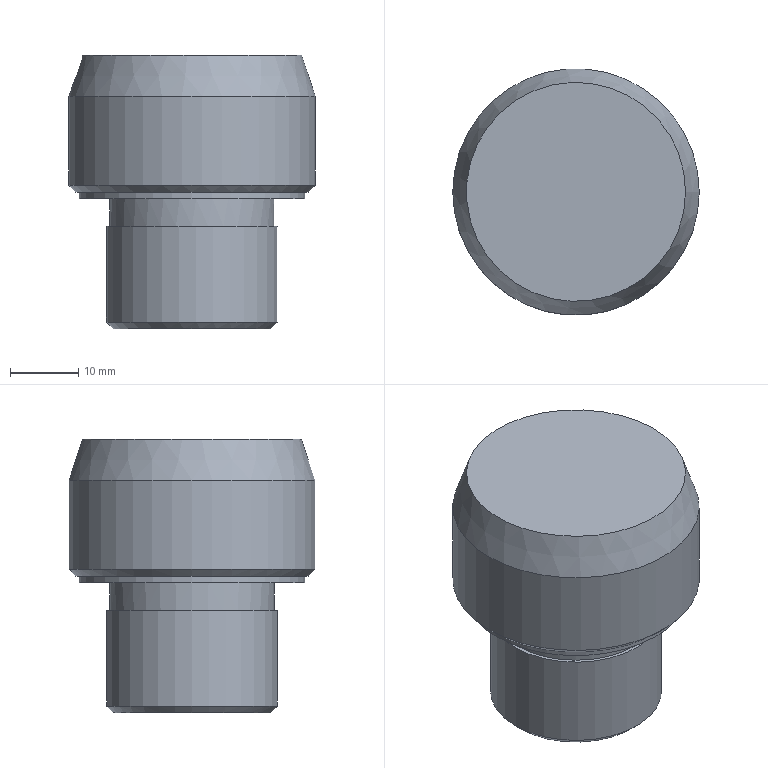Component | NX | CYL_LOC_PIN | 1 solid | 12 faces | box 36 x 36 x 40 mm | volume 29638 mm3 | plane 5 | cylinder 4 | cone 3 | commonest cylinder face diameters 36 x1 33 x1 24 x1 25 x1
STEP:
#1=CARTESIAN_POINT('',(0.,0.,0.));
#2=DIRECTION('',(0.,0.,1.));
#3=DIRECTION('',(1.,0.,0.));
#4=AXIS2_PLACEMENT_3D('',#1,#2,#3);
#5=CARTESIAN_POINT('',(-105.,0.,-236.));
#6=VERTEX_POINT('',#5);
#7=CARTESIAN_POINT('',(-88.,0.,-236.));
#8=DIRECTION('',(0.,0.,-1.));
#9=DIRECTION('',(-1.,0.,0.));
#10=AXIS2_PLACEMENT_3D('',#7,#8,#9);
#11=CIRCLE('',#10,17.);
#12=CARTESIAN_POINT('',(-88.,0.,-236.));
#13=DIRECTION('',(0.,0.,-1.));
#14=DIRECTION('',(-1.,0.,0.));
#15=AXIS2_PLACEMENT_3D('',#12,#13,#14);
#16=PLANE('',#15);
#17=CARTESIAN_POINT('',(0.,0.));
#18=DIRECTION('',(1.,0.));
#19=AXIS2_PLACEMENT_2D('',#17,#18);
#20=CIRCLE('',#19,17.);
#21=(GEOMETRIC_REPRESENTATION_CONTEXT(2)PARAMETRIC_REPRESENTATION_CONTEXT()REPRESENTATION_CONTEXT('',''));
#22=DEFINITIONAL_REPRESENTATION('',(#20),#21);
#23=PCURVE('',#16,#22);
#24=CARTESIAN_POINT('',(-88.,0.,-235.));
#25=DIRECTION('',(0.,0.,1.));
#26=DIRECTION('',(1.,0.,0.));
#27=AXIS2_PLACEMENT_3D('',#24,#25,#26);
#28=CONICAL_SURFACE('',#27,18.,0.7854);
#29=CARTESIAN_POINT('',(9.425,-1.));
#30=DIRECTION('',(-1.,0.));
#31=VECTOR('',#30,1.);
#32=LINE('',#29,#31);
#33=(GEOMETRIC_REPRESENTATION_CONTEXT(2)PARAMETRIC_REPRESENTATION_CONTEXT()REPRESENTATION_CONTEXT('',''));
#34=DEFINITIONAL_REPRESENTATION('',(#32),#33);
#35=PCURVE('',#28,#34);
#36=SURFACE_CURVE('',#11,(#23,#35),.PCURVE_S1.);
#37=EDGE_CURVE('',#6,#6,#36,.T.);
#38=ORIENTED_EDGE('',*,*,#37,.T.);
#39=EDGE_LOOP('',(#38));
#40=FACE_BOUND('',#39,.T.);
#41=CARTESIAN_POINT('',(-104.5,0.,-236.));
#42=VERTEX_POINT('',#41);
#43=CARTESIAN_POINT('',(-88.,0.,-236.));
#44=DIRECTION('',(0.,0.,-1.));
#45=DIRECTION('',(-1.,0.,0.));
#46=AXIS2_PLACEMENT_3D('',#43,#44,#45);
#47=CIRCLE('',#46,16.5);
#48=CARTESIAN_POINT('',(0.,0.));
#49=DIRECTION('',(1.,0.));
#50=AXIS2_PLACEMENT_2D('',#48,#49);
#51=CIRCLE('',#50,16.5);
#52=(GEOMETRIC_REPRESENTATION_CONTEXT(2)PARAMETRIC_REPRESENTATION_CONTEXT()REPRESENTATION_CONTEXT('',''));
#53=DEFINITIONAL_REPRESENTATION('',(#51),#52);
#54=PCURVE('',#16,#53);
#55=CARTESIAN_POINT('',(-88.,0.,-236.));
#56=DIRECTION('',(0.,0.,-1.));
#57=DIRECTION('',(-1.,0.,0.));
#58=AXIS2_PLACEMENT_3D('',#55,#56,#57);
#59=CYLINDRICAL_SURFACE('',#58,16.5);
#60=CARTESIAN_POINT('',(0.,0.));
#61=DIRECTION('',(1.,0.));
#62=VECTOR('',#61,1.);
#63=LINE('',#60,#62);
#64=(GEOMETRIC_REPRESENTATION_CONTEXT(2)PARAMETRIC_REPRESENTATION_CONTEXT()REPRESENTATION_CONTEXT('',''));
#65=DEFINITIONAL_REPRESENTATION('',(#63),#64);
#66=PCURVE('',#59,#65);
#67=SURFACE_CURVE('',#47,(#54,#66),.PCURVE_S1.);
#68=EDGE_CURVE('',#42,#42,#67,.T.);
#69=ORIENTED_EDGE('',*,*,#68,.F.);
#70=EDGE_LOOP('',(#69));
#71=FACE_BOUND('',#70,.T.);
#72=ADVANCED_FACE('',(#40,#71),#16,.T.);
#73=CARTESIAN_POINT('',(-72.,0.,-216.));
#74=VERTEX_POINT('',#73);
#75=CARTESIAN_POINT('',(-88.,0.,-216.));
#76=DIRECTION('',(0.,0.,1.));
#77=DIRECTION('',(1.,0.,0.));
#78=AXIS2_PLACEMENT_3D('',#75,#76,#77);
#79=CIRCLE('',#78,16.);
#80=CARTESIAN_POINT('',(-88.,0.,-216.));
#81=DIRECTION('',(0.,0.,1.));
#82=DIRECTION('',(1.,0.,0.));
#83=AXIS2_PLACEMENT_3D('',#80,#81,#82);
#84=PLANE('',#83);
#85=CARTESIAN_POINT('',(0.,0.));
#86=DIRECTION('',(1.,0.));
#87=AXIS2_PLACEMENT_2D('',#85,#86);
#88=CIRCLE('',#87,16.);
#89=(GEOMETRIC_REPRESENTATION_CONTEXT(2)PARAMETRIC_REPRESENTATION_CONTEXT()REPRESENTATION_CONTEXT('',''));
#90=DEFINITIONAL_REPRESENTATION('',(#88),#89);
#91=PCURVE('',#84,#90);
#92=CARTESIAN_POINT('',(-88.,0.,-222.));
#93=DIRECTION('',(0.,0.,-1.));
#94=DIRECTION('',(-1.,0.,0.));
#95=AXIS2_PLACEMENT_3D('',#92,#93,#94);
#96=CONICAL_SURFACE('',#95,18.,0.3218);
#97=CARTESIAN_POINT('',(9.425,-6.));
#98=DIRECTION('',(-1.,0.));
#99=VECTOR('',#98,1.);
#100=LINE('',#97,#99);
#101=(GEOMETRIC_REPRESENTATION_CONTEXT(2)PARAMETRIC_REPRESENTATION_CONTEXT()REPRESENTATION_CONTEXT('',''));
#102=DEFINITIONAL_REPRESENTATION('',(#100),#101);
#103=PCURVE('',#96,#102);
#104=SURFACE_CURVE('',#79,(#91,#103),.PCURVE_S1.);
#105=EDGE_CURVE('',#74,#74,#104,.T.);
#106=ORIENTED_EDGE('',*,*,#105,.T.);
#107=EDGE_LOOP('',(#106));
#108=FACE_BOUND('',#107,.T.);
#109=ADVANCED_FACE('',(#108),#84,.T.);
#110=CARTESIAN_POINT('',(-106.,0.,-235.));
#111=VERTEX_POINT('',#110);
#112=CARTESIAN_POINT('',(-88.,0.,-235.));
#113=DIRECTION('',(0.,0.,1.));
#114=DIRECTION('',(-1.,0.,0.));
#115=AXIS2_PLACEMENT_3D('',#112,#113,#114);
#116=CIRCLE('',#115,18.);
#117=CARTESIAN_POINT('',(-88.,0.,-216.));
#118=DIRECTION('',(0.,0.,-1.));
#119=DIRECTION('',(-1.,0.,0.));
#120=AXIS2_PLACEMENT_3D('',#117,#118,#119);
#121=CYLINDRICAL_SURFACE('',#120,18.);
#122=CARTESIAN_POINT('',(6.283,19.));
#123=DIRECTION('',(-1.,0.));
#124=VECTOR('',#123,1.);
#125=LINE('',#122,#124);
#126=(GEOMETRIC_REPRESENTATION_CONTEXT(2)PARAMETRIC_REPRESENTATION_CONTEXT()REPRESENTATION_CONTEXT('',''));
#127=DEFINITIONAL_REPRESENTATION('',(#125),#126);
#128=PCURVE('',#121,#127);
#129=CARTESIAN_POINT('',(3.142,0.));
#130=DIRECTION('',(1.,0.));
#131=VECTOR('',#130,1.);
#132=LINE('',#129,#131);
#133=(GEOMETRIC_REPRESENTATION_CONTEXT(2)PARAMETRIC_REPRESENTATION_CONTEXT()REPRESENTATION_CONTEXT('',''));
#134=DEFINITIONAL_REPRESENTATION('',(#132),#133);
#135=PCURVE('',#28,#134);
#136=SURFACE_CURVE('',#116,(#128,#135),.PCURVE_S1.);
#137=EDGE_CURVE('',#111,#111,#136,.T.);
#138=ORIENTED_EDGE('',*,*,#137,.T.);
#139=CARTESIAN_POINT('',(-106.,0.,-222.));
#140=VERTEX_POINT('',#139);
#141=CARTESIAN_POINT('',(-106.,0.,-222.));
#142=CARTESIAN_POINT('',(-106.,0.,-235.));
#143=B_SPLINE_CURVE_WITH_KNOTS('',1,(#141,#142),.UNSPECIFIED.,.F.,.F.,(2,2),(6.,19.),.PIECEWISE_BEZIER_KNOTS.);
#144=CARTESIAN_POINT('',(0.,0.));
#145=DIRECTION('',(0.,1.));
#146=VECTOR('',#145,1.);
#147=LINE('',#144,#146);
#148=(GEOMETRIC_REPRESENTATION_CONTEXT(2)PARAMETRIC_REPRESENTATION_CONTEXT()REPRESENTATION_CONTEXT('',''));
#149=DEFINITIONAL_REPRESENTATION('',(#147),#148);
#150=PCURVE('',#121,#149);
#151=CARTESIAN_POINT('',(6.283,0.));
#152=DIRECTION('',(0.,1.));
#153=VECTOR('',#152,1.);
#154=LINE('',#151,#153);
#155=(GEOMETRIC_REPRESENTATION_CONTEXT(2)PARAMETRIC_REPRESENTATION_CONTEXT()REPRESENTATION_CONTEXT('',''));
#156=DEFINITIONAL_REPRESENTATION('',(#154),#155);
#157=PCURVE('',#121,#156);
#158=SEAM_CURVE('',#143,(#150,#157),.PCURVE_S1.);
#159=EDGE_CURVE('',#140,#111,#158,.T.);
#160=ORIENTED_EDGE('',*,*,#159,.F.);
#161=CARTESIAN_POINT('',(-70.,0.,-222.));
#162=VERTEX_POINT('',#161);
#163=CARTESIAN_POINT('',(-88.,0.,-222.));
#164=DIRECTION('',(0.,0.,-1.));
#165=DIRECTION('',(1.,0.,0.));
#166=AXIS2_PLACEMENT_3D('',#163,#164,#165);
#167=CIRCLE('',#166,18.);
#168=CARTESIAN_POINT('',(-3.142,6.));
#169=DIRECTION('',(1.,0.));
#170=VECTOR('',#169,1.);
#171=LINE('',#168,#170);
#172=(GEOMETRIC_REPRESENTATION_CONTEXT(2)PARAMETRIC_REPRESENTATION_CONTEXT()REPRESENTATION_CONTEXT('',''));
#173=DEFINITIONAL_REPRESENTATION('',(#171),#172);
#174=PCURVE('',#121,#173);
#175=CARTESIAN_POINT('',(3.142,0.));
#176=DIRECTION('',(1.,0.));
#177=VECTOR('',#176,1.);
#178=LINE('',#175,#177);
#179=(GEOMETRIC_REPRESENTATION_CONTEXT(2)PARAMETRIC_REPRESENTATION_CONTEXT()REPRESENTATION_CONTEXT('',''));
#180=DEFINITIONAL_REPRESENTATION('',(#178),#179);
#181=PCURVE('',#96,#180);
#182=SURFACE_CURVE('',#167,(#174,#181),.PCURVE_S1.);
#183=EDGE_CURVE('',#140,#162,#182,.T.);
#184=ORIENTED_EDGE('',*,*,#183,.T.);
#185=CARTESIAN_POINT('',(-88.,0.,-222.));
#186=DIRECTION('',(0.,0.,-1.));
#187=DIRECTION('',(1.,0.,0.));
#188=AXIS2_PLACEMENT_3D('',#185,#186,#187);
#189=CIRCLE('',#188,18.);
#190=CARTESIAN_POINT('',(3.142,6.));
#191=DIRECTION('',(1.,0.));
#192=VECTOR('',#191,1.);
#193=LINE('',#190,#192);
#194=(GEOMETRIC_REPRESENTATION_CONTEXT(2)PARAMETRIC_REPRESENTATION_CONTEXT()REPRESENTATION_CONTEXT('',''));
#195=DEFINITIONAL_REPRESENTATION('',(#193),#194);
#196=PCURVE('',#121,#195);
#197=CARTESIAN_POINT('',(3.142,0.));
#198=DIRECTION('',(1.,0.));
#199=VECTOR('',#198,1.);
#200=LINE('',#197,#199);
#201=(GEOMETRIC_REPRESENTATION_CONTEXT(2)PARAMETRIC_REPRESENTATION_CONTEXT()REPRESENTATION_CONTEXT('',''));
#202=DEFINITIONAL_REPRESENTATION('',(#200),#201);
#203=PCURVE('',#96,#202);
#204=SURFACE_CURVE('',#189,(#196,#203),.PCURVE_S1.);
#205=EDGE_CURVE('',#162,#140,#204,.T.);
#206=ORIENTED_EDGE('',*,*,#205,.T.);
#207=ORIENTED_EDGE('',*,*,#159,.T.);
#208=EDGE_LOOP('',(#138,#160,#184,#206,#207));
#209=FACE_BOUND('',#208,.T.);
#210=ADVANCED_FACE('',(#209),#121,.T.);
#211=CARTESIAN_POINT('',(-100.,0.,-237.));
#212=VERTEX_POINT('',#211);
#213=CARTESIAN_POINT('',(-88.,0.,-237.));
#214=DIRECTION('',(0.,0.,-1.));
#215=DIRECTION('',(-1.,0.,0.));
#216=AXIS2_PLACEMENT_3D('',#213,#214,#215);
#217=CIRCLE('',#216,12.);
#218=CARTESIAN_POINT('',(-88.,0.,-237.));
#219=DIRECTION('',(0.,0.,-1.));
#220=DIRECTION('',(-1.,0.,0.));
#221=AXIS2_PLACEMENT_3D('',#218,#219,#220);
#222=PLANE('',#221);
#223=CARTESIAN_POINT('',(0.,0.));
#224=DIRECTION('',(1.,0.));
#225=AXIS2_PLACEMENT_2D('',#223,#224);
#226=CIRCLE('',#225,12.);
#227=(GEOMETRIC_REPRESENTATION_CONTEXT(2)PARAMETRIC_REPRESENTATION_CONTEXT()REPRESENTATION_CONTEXT('',''));
#228=DEFINITIONAL_REPRESENTATION('',(#226),#227);
#229=PCURVE('',#222,#228);
#230=CARTESIAN_POINT('',(-88.,0.,-237.));
#231=DIRECTION('',(0.,0.,-1.));
#232=DIRECTION('',(-1.,0.,0.));
#233=AXIS2_PLACEMENT_3D('',#230,#231,#232);
#234=CYLINDRICAL_SURFACE('',#233,12.);
#235=CARTESIAN_POINT('',(0.,0.));
#236=DIRECTION('',(1.,0.));
#237=VECTOR('',#236,1.);
#238=LINE('',#235,#237);
#239=(GEOMETRIC_REPRESENTATION_CONTEXT(2)PARAMETRIC_REPRESENTATION_CONTEXT()REPRESENTATION_CONTEXT('',''));
#240=DEFINITIONAL_REPRESENTATION('',(#238),#239);
#241=PCURVE('',#234,#240);
#242=SURFACE_CURVE('',#217,(#229,#241),.PCURVE_S1.);
#243=EDGE_CURVE('',#212,#212,#242,.T.);
#244=ORIENTED_EDGE('',*,*,#243,.F.);
#245=EDGE_LOOP('',(#244));
#246=FACE_BOUND('',#245,.T.);
#247=CARTESIAN_POINT('',(-104.5,0.,-237.));
#248=VERTEX_POINT('',#247);
#249=CARTESIAN_POINT('',(-88.,0.,-237.));
#250=DIRECTION('',(0.,0.,1.));
#251=DIRECTION('',(-1.,0.,0.));
#252=AXIS2_PLACEMENT_3D('',#249,#250,#251);
#253=CIRCLE('',#252,16.5);
#254=CARTESIAN_POINT('',(16.5,0.));
#255=CARTESIAN_POINT('',(16.5,-28.579));
#256=CARTESIAN_POINT('',(-8.25,-14.289));
#257=CARTESIAN_POINT('',(-33.,-0.));
#258=CARTESIAN_POINT('',(-8.25,14.289));
#259=CARTESIAN_POINT('',(16.5,28.579));
#260=CARTESIAN_POINT('',(16.5,0.));
#261=(BOUNDED_CURVE()B_SPLINE_CURVE(2,(#254,#255,#256,#257,#258,#259,#260),.UNSPECIFIED.,.T.,.F.)B_SPLINE_CURVE_WITH_KNOTS((1,2,2,2,2,1),(-2.094,0.,2.094,4.189,6.283,8.378),.UNSPECIFIED.)CURVE()GEOMETRIC_REPRESENTATION_ITEM()RATIONAL_B_SPLINE_CURVE((1.,0.5,1.,0.5,1.,0.5,1.))REPRESENTATION_ITEM(''));
#262=(GEOMETRIC_REPRESENTATION_CONTEXT(2)PARAMETRIC_REPRESENTATION_CONTEXT()REPRESENTATION_CONTEXT('',''));
#263=DEFINITIONAL_REPRESENTATION('',(#261),#262);
#264=PCURVE('',#222,#263);
#265=CARTESIAN_POINT('',(6.283,1.));
#266=DIRECTION('',(-1.,0.));
#267=VECTOR('',#266,1.);
#268=LINE('',#265,#267);
#269=(GEOMETRIC_REPRESENTATION_CONTEXT(2)PARAMETRIC_REPRESENTATION_CONTEXT()REPRESENTATION_CONTEXT('',''));
#270=DEFINITIONAL_REPRESENTATION('',(#268),#269);
#271=PCURVE('',#59,#270);
#272=SURFACE_CURVE('',#253,(#264,#271),.PCURVE_S1.);
#273=EDGE_CURVE('',#248,#248,#272,.T.);
#274=ORIENTED_EDGE('',*,*,#273,.F.);
#275=EDGE_LOOP('',(#274));
#276=FACE_BOUND('',#275,.T.);
#277=ADVANCED_FACE('',(#246,#276),#222,.T.);
#278=ORIENTED_EDGE('',*,*,#273,.T.);
#279=CARTESIAN_POINT('',(-104.5,0.,-236.));
#280=CARTESIAN_POINT('',(-104.5,0.,-237.));
#281=B_SPLINE_CURVE_WITH_KNOTS('',1,(#279,#280),.UNSPECIFIED.,.F.,.F.,(2,2),(0.,1.),.PIECEWISE_BEZIER_KNOTS.);
#282=CARTESIAN_POINT('',(0.,0.));
#283=DIRECTION('',(0.,1.));
#284=VECTOR('',#283,1.);
#285=LINE('',#282,#284);
#286=(GEOMETRIC_REPRESENTATION_CONTEXT(2)PARAMETRIC_REPRESENTATION_CONTEXT()REPRESENTATION_CONTEXT('',''));
#287=DEFINITIONAL_REPRESENTATION('',(#285),#286);
#288=PCURVE('',#59,#287);
#289=CARTESIAN_POINT('',(6.283,0.));
#290=DIRECTION('',(0.,1.));
#291=VECTOR('',#290,1.);
#292=LINE('',#289,#291);
#293=(GEOMETRIC_REPRESENTATION_CONTEXT(2)PARAMETRIC_REPRESENTATION_CONTEXT()REPRESENTATION_CONTEXT('',''));
#294=DEFINITIONAL_REPRESENTATION('',(#292),#293);
#295=PCURVE('',#59,#294);
#296=SEAM_CURVE('',#281,(#288,#295),.PCURVE_S1.);
#297=EDGE_CURVE('',#42,#248,#296,.T.);
#298=ORIENTED_EDGE('',*,*,#297,.F.);
#299=ORIENTED_EDGE('',*,*,#68,.T.);
#300=ORIENTED_EDGE('',*,*,#297,.T.);
#301=EDGE_LOOP('',(#278,#298,#299,#300));
#302=FACE_BOUND('',#301,.T.);
#303=ADVANCED_FACE('',(#302),#59,.T.);
#304=CARTESIAN_POINT('',(-100.,0.,-241.));
#305=VERTEX_POINT('',#304);
#306=CARTESIAN_POINT('',(-76.,0.,-241.));
#307=VERTEX_POINT('',#306);
#308=CARTESIAN_POINT('',(-88.,0.,-241.));
#309=DIRECTION('',(0.,0.,-1.));
#310=DIRECTION('',(1.,0.,0.));
#311=AXIS2_PLACEMENT_3D('',#308,#309,#310);
#312=CIRCLE('',#311,12.);
#313=CARTESIAN_POINT('',(-3.142,4.));
#314=DIRECTION('',(1.,0.));
#315=VECTOR('',#314,1.);
#316=LINE('',#313,#315);
#317=(GEOMETRIC_REPRESENTATION_CONTEXT(2)PARAMETRIC_REPRESENTATION_CONTEXT()REPRESENTATION_CONTEXT('',''));
#318=DEFINITIONAL_REPRESENTATION('',(#316),#317);
#319=PCURVE('',#234,#318);
#320=CARTESIAN_POINT('',(-88.,0.,-241.));
#321=DIRECTION('',(0.,0.,1.));
#322=DIRECTION('',(1.,0.,0.));
#323=AXIS2_PLACEMENT_3D('',#320,#321,#322);
#324=PLANE('',#323);
#325=CARTESIAN_POINT('',(12.,0.));
#326=CARTESIAN_POINT('',(12.,-20.785));
#327=CARTESIAN_POINT('',(-6.,-10.392));
#328=CARTESIAN_POINT('',(-24.,-0.));
#329=CARTESIAN_POINT('',(-6.,10.392));
#330=CARTESIAN_POINT('',(12.,20.785));
#331=CARTESIAN_POINT('',(12.,0.));
#332=(BOUNDED_CURVE()B_SPLINE_CURVE(2,(#325,#326,#327,#328,#329,#330,#331),.UNSPECIFIED.,.T.,.F.)B_SPLINE_CURVE_WITH_KNOTS((1,2,2,2,2,1),(-2.094,0.,2.094,4.189,6.283,8.378),.UNSPECIFIED.)CURVE()GEOMETRIC_REPRESENTATION_ITEM()RATIONAL_B_SPLINE_CURVE((1.,0.5,1.,0.5,1.,0.5,1.))REPRESENTATION_ITEM(''));
#333=(GEOMETRIC_REPRESENTATION_CONTEXT(2)PARAMETRIC_REPRESENTATION_CONTEXT()REPRESENTATION_CONTEXT('',''));
#334=DEFINITIONAL_REPRESENTATION('',(#332),#333);
#335=PCURVE('',#324,#334);
#336=SURFACE_CURVE('',#312,(#319,#335),.PCURVE_S1.);
#337=EDGE_CURVE('',#305,#307,#336,.T.);
#338=ORIENTED_EDGE('',*,*,#337,.F.);
#339=CARTESIAN_POINT('',(-100.,0.,-237.));
#340=CARTESIAN_POINT('',(-100.,0.,-241.));
#341=B_SPLINE_CURVE_WITH_KNOTS('',1,(#339,#340),.UNSPECIFIED.,.F.,.F.,(2,2),(0.,4.),.PIECEWISE_BEZIER_KNOTS.);
#342=CARTESIAN_POINT('',(0.,0.));
#343=DIRECTION('',(0.,1.));
#344=VECTOR('',#343,1.);
#345=LINE('',#342,#344);
#346=(GEOMETRIC_REPRESENTATION_CONTEXT(2)PARAMETRIC_REPRESENTATION_CONTEXT()REPRESENTATION_CONTEXT('',''));
#347=DEFINITIONAL_REPRESENTATION('',(#345),#346);
#348=PCURVE('',#234,#347);
#349=CARTESIAN_POINT('',(6.283,0.));
#350=DIRECTION('',(0.,1.));
#351=VECTOR('',#350,1.);
#352=LINE('',#349,#351);
#353=(GEOMETRIC_REPRESENTATION_CONTEXT(2)PARAMETRIC_REPRESENTATION_CONTEXT()REPRESENTATION_CONTEXT('',''));
#354=DEFINITIONAL_REPRESENTATION('',(#352),#353);
#355=PCURVE('',#234,#354);
#356=SEAM_CURVE('',#341,(#348,#355),.PCURVE_S1.);
#357=EDGE_CURVE('',#212,#305,#356,.T.);
#358=ORIENTED_EDGE('',*,*,#357,.F.);
#359=ORIENTED_EDGE('',*,*,#243,.T.);
#360=ORIENTED_EDGE('',*,*,#357,.T.);
#361=CARTESIAN_POINT('',(-88.,0.,-241.));
#362=DIRECTION('',(0.,0.,-1.));
#363=DIRECTION('',(1.,0.,0.));
#364=AXIS2_PLACEMENT_3D('',#361,#362,#363);
#365=CIRCLE('',#364,12.);
#366=CARTESIAN_POINT('',(3.142,4.));
#367=DIRECTION('',(1.,0.));
#368=VECTOR('',#367,1.);
#369=LINE('',#366,#368);
#370=(GEOMETRIC_REPRESENTATION_CONTEXT(2)PARAMETRIC_REPRESENTATION_CONTEXT()REPRESENTATION_CONTEXT('',''));
#371=DEFINITIONAL_REPRESENTATION('',(#369),#370);
#372=PCURVE('',#234,#371);
#373=CARTESIAN_POINT('',(12.,0.));
#374=CARTESIAN_POINT('',(12.,-20.785));
#375=CARTESIAN_POINT('',(-6.,-10.392));
#376=CARTESIAN_POINT('',(-24.,-0.));
#377=CARTESIAN_POINT('',(-6.,10.392));
#378=CARTESIAN_POINT('',(12.,20.785));
#379=CARTESIAN_POINT('',(12.,0.));
#380=(BOUNDED_CURVE()B_SPLINE_CURVE(2,(#373,#374,#375,#376,#377,#378,#379),.UNSPECIFIED.,.T.,.F.)B_SPLINE_CURVE_WITH_KNOTS((1,2,2,2,2,1),(-2.094,0.,2.094,4.189,6.283,8.378),.UNSPECIFIED.)CURVE()GEOMETRIC_REPRESENTATION_ITEM()RATIONAL_B_SPLINE_CURVE((1.,0.5,1.,0.5,1.,0.5,1.))REPRESENTATION_ITEM(''));
#381=(GEOMETRIC_REPRESENTATION_CONTEXT(2)PARAMETRIC_REPRESENTATION_CONTEXT()REPRESENTATION_CONTEXT('',''));
#382=DEFINITIONAL_REPRESENTATION('',(#380),#381);
#383=PCURVE('',#324,#382);
#384=SURFACE_CURVE('',#365,(#372,#383),.PCURVE_S1.);
#385=EDGE_CURVE('',#307,#305,#384,.T.);
#386=ORIENTED_EDGE('',*,*,#385,.F.);
#387=EDGE_LOOP('',(#338,#358,#359,#360,#386));
#388=FACE_BOUND('',#387,.T.);
#389=ADVANCED_FACE('',(#388),#234,.T.);
#390=CARTESIAN_POINT('',(-99.5,0.,-256.));
#391=VERTEX_POINT('',#390);
#392=CARTESIAN_POINT('',(-88.,0.,-256.));
#393=DIRECTION('',(0.,0.,-1.));
#394=DIRECTION('',(-1.,0.,0.));
#395=AXIS2_PLACEMENT_3D('',#392,#393,#394);
#396=CIRCLE('',#395,11.5);
#397=CARTESIAN_POINT('',(-88.,0.,-256.));
#398=DIRECTION('',(0.,0.,-1.));
#399=DIRECTION('',(-1.,0.,0.));
#400=AXIS2_PLACEMENT_3D('',#397,#398,#399);
#401=PLANE('',#400);
#402=CARTESIAN_POINT('',(0.,0.));
#403=DIRECTION('',(1.,0.));
#404=AXIS2_PLACEMENT_2D('',#402,#403);
#405=CIRCLE('',#404,11.5);
#406=(GEOMETRIC_REPRESENTATION_CONTEXT(2)PARAMETRIC_REPRESENTATION_CONTEXT()REPRESENTATION_CONTEXT('',''));
#407=DEFINITIONAL_REPRESENTATION('',(#405),#406);
#408=PCURVE('',#401,#407);
#409=CARTESIAN_POINT('',(-88.,0.,-255.));
#410=DIRECTION('',(0.,0.,1.));
#411=DIRECTION('',(1.,0.,0.));
#412=AXIS2_PLACEMENT_3D('',#409,#410,#411);
#413=CONICAL_SURFACE('',#412,12.5,0.7854);
#414=CARTESIAN_POINT('',(9.425,-1.));
#415=DIRECTION('',(-1.,0.));
#416=VECTOR('',#415,1.);
#417=LINE('',#414,#416);
#418=(GEOMETRIC_REPRESENTATION_CONTEXT(2)PARAMETRIC_REPRESENTATION_CONTEXT()REPRESENTATION_CONTEXT('',''));
#419=DEFINITIONAL_REPRESENTATION('',(#417),#418);
#420=PCURVE('',#413,#419);
#421=SURFACE_CURVE('',#396,(#408,#420),.PCURVE_S1.);
#422=EDGE_CURVE('',#391,#391,#421,.T.);
#423=ORIENTED_EDGE('',*,*,#422,.T.);
#424=EDGE_LOOP('',(#423));
#425=FACE_BOUND('',#424,.T.);
#426=ADVANCED_FACE('',(#425),#401,.T.);
#427=ORIENTED_EDGE('',*,*,#385,.T.);
#428=ORIENTED_EDGE('',*,*,#337,.T.);
#429=EDGE_LOOP('',(#427,#428));
#430=FACE_BOUND('',#429,.T.);
#431=CARTESIAN_POINT('',(-100.5,0.,-241.));
#432=VERTEX_POINT('',#431);
#433=CARTESIAN_POINT('',(-88.,0.,-241.));
#434=DIRECTION('',(0.,0.,-1.));
#435=DIRECTION('',(-1.,0.,0.));
#436=AXIS2_PLACEMENT_3D('',#433,#434,#435);
#437=CIRCLE('',#436,12.5);
#438=CARTESIAN_POINT('',(-12.5,0.));
#439=CARTESIAN_POINT('',(-12.5,21.651));
#440=CARTESIAN_POINT('',(6.25,10.825));
#441=CARTESIAN_POINT('',(25.,0.));
#442=CARTESIAN_POINT('',(6.25,-10.825));
#443=CARTESIAN_POINT('',(-12.5,-21.651));
#444=CARTESIAN_POINT('',(-12.5,0.));
#445=(BOUNDED_CURVE()B_SPLINE_CURVE(2,(#438,#439,#440,#441,#442,#443,#444),.UNSPECIFIED.,.T.,.F.)B_SPLINE_CURVE_WITH_KNOTS((1,2,2,2,2,1),(-2.094,0.,2.094,4.189,6.283,8.378),.UNSPECIFIED.)CURVE()GEOMETRIC_REPRESENTATION_ITEM()RATIONAL_B_SPLINE_CURVE((1.,0.5,1.,0.5,1.,0.5,1.))REPRESENTATION_ITEM(''));
#446=(GEOMETRIC_REPRESENTATION_CONTEXT(2)PARAMETRIC_REPRESENTATION_CONTEXT()REPRESENTATION_CONTEXT('',''));
#447=DEFINITIONAL_REPRESENTATION('',(#445),#446);
#448=PCURVE('',#324,#447);
#449=CARTESIAN_POINT('',(-88.,0.,-241.));
#450=DIRECTION('',(0.,0.,-1.));
#451=DIRECTION('',(-1.,0.,0.));
#452=AXIS2_PLACEMENT_3D('',#449,#450,#451);
#453=CYLINDRICAL_SURFACE('',#452,12.5);
#454=CARTESIAN_POINT('',(0.,0.));
#455=DIRECTION('',(1.,0.));
#456=VECTOR('',#455,1.);
#457=LINE('',#454,#456);
#458=(GEOMETRIC_REPRESENTATION_CONTEXT(2)PARAMETRIC_REPRESENTATION_CONTEXT()REPRESENTATION_CONTEXT('',''));
#459=DEFINITIONAL_REPRESENTATION('',(#457),#458);
#460=PCURVE('',#453,#459);
#461=SURFACE_CURVE('',#437,(#448,#460),.PCURVE_S1.);
#462=EDGE_CURVE('',#432,#432,#461,.T.);
#463=ORIENTED_EDGE('',*,*,#462,.F.);
#464=EDGE_LOOP('',(#463));
#465=FACE_BOUND('',#464,.T.);
#466=ADVANCED_FACE('',(#430,#465),#324,.T.);
#467=CARTESIAN_POINT('',(-100.5,0.,-255.));
#468=VERTEX_POINT('',#467);
#469=CARTESIAN_POINT('',(-88.,0.,-255.));
#470=DIRECTION('',(0.,0.,1.));
#471=DIRECTION('',(-1.,0.,0.));
#472=AXIS2_PLACEMENT_3D('',#469,#470,#471);
#473=CIRCLE('',#472,12.5);
#474=CARTESIAN_POINT('',(6.283,14.));
#475=DIRECTION('',(-1.,0.));
#476=VECTOR('',#475,1.);
#477=LINE('',#474,#476);
#478=(GEOMETRIC_REPRESENTATION_CONTEXT(2)PARAMETRIC_REPRESENTATION_CONTEXT()REPRESENTATION_CONTEXT('',''));
#479=DEFINITIONAL_REPRESENTATION('',(#477),#478);
#480=PCURVE('',#453,#479);
#481=CARTESIAN_POINT('',(3.142,0.));
#482=DIRECTION('',(1.,0.));
#483=VECTOR('',#482,1.);
#484=LINE('',#481,#483);
#485=(GEOMETRIC_REPRESENTATION_CONTEXT(2)PARAMETRIC_REPRESENTATION_CONTEXT()REPRESENTATION_CONTEXT('',''));
#486=DEFINITIONAL_REPRESENTATION('',(#484),#485);
#487=PCURVE('',#413,#486);
#488=SURFACE_CURVE('',#473,(#480,#487),.PCURVE_S1.);
#489=EDGE_CURVE('',#468,#468,#488,.T.);
#490=ORIENTED_EDGE('',*,*,#489,.T.);
#491=CARTESIAN_POINT('',(-100.5,0.,-241.));
#492=CARTESIAN_POINT('',(-100.5,0.,-255.));
#493=B_SPLINE_CURVE_WITH_KNOTS('',1,(#491,#492),.UNSPECIFIED.,.F.,.F.,(2,2),(0.,14.),.PIECEWISE_BEZIER_KNOTS.);
#494=CARTESIAN_POINT('',(0.,0.));
#495=DIRECTION('',(0.,1.));
#496=VECTOR('',#495,1.);
#497=LINE('',#494,#496);
#498=(GEOMETRIC_REPRESENTATION_CONTEXT(2)PARAMETRIC_REPRESENTATION_CONTEXT()REPRESENTATION_CONTEXT('',''));
#499=DEFINITIONAL_REPRESENTATION('',(#497),#498);
#500=PCURVE('',#453,#499);
#501=CARTESIAN_POINT('',(6.283,0.));
#502=DIRECTION('',(0.,1.));
#503=VECTOR('',#502,1.);
#504=LINE('',#501,#503);
#505=(GEOMETRIC_REPRESENTATION_CONTEXT(2)PARAMETRIC_REPRESENTATION_CONTEXT()REPRESENTATION_CONTEXT('',''));
#506=DEFINITIONAL_REPRESENTATION('',(#504),#505);
#507=PCURVE('',#453,#506);
#508=SEAM_CURVE('',#493,(#500,#507),.PCURVE_S1.);
#509=EDGE_CURVE('',#432,#468,#508,.T.);
#510=ORIENTED_EDGE('',*,*,#509,.F.);
#511=ORIENTED_EDGE('',*,*,#462,.T.);
#512=ORIENTED_EDGE('',*,*,#509,.T.);
#513=EDGE_LOOP('',(#490,#510,#511,#512));
#514=FACE_BOUND('',#513,.T.);
#515=ADVANCED_FACE('',(#514),#453,.T.);
#516=ORIENTED_EDGE('',*,*,#105,.F.);
#517=CARTESIAN_POINT('',(-72.,0.,-216.));
#518=CARTESIAN_POINT('',(-70.,0.,-222.));
#519=B_SPLINE_CURVE_WITH_KNOTS('',1,(#517,#518),.UNSPECIFIED.,.F.,.F.,(2,2),(-6.325,0.),.PIECEWISE_BEZIER_KNOTS.);
#520=CARTESIAN_POINT('',(9.425,0.));
#521=DIRECTION('',(0.,1.));
#522=VECTOR('',#521,1.);
#523=LINE('',#520,#522);
#524=(GEOMETRIC_REPRESENTATION_CONTEXT(2)PARAMETRIC_REPRESENTATION_CONTEXT()REPRESENTATION_CONTEXT('',''));
#525=DEFINITIONAL_REPRESENTATION('',(#523),#524);
#526=PCURVE('',#96,#525);
#527=CARTESIAN_POINT('',(3.142,0.));
#528=DIRECTION('',(0.,1.));
#529=VECTOR('',#528,1.);
#530=LINE('',#527,#529);
#531=(GEOMETRIC_REPRESENTATION_CONTEXT(2)PARAMETRIC_REPRESENTATION_CONTEXT()REPRESENTATION_CONTEXT('',''));
#532=DEFINITIONAL_REPRESENTATION('',(#530),#531);
#533=PCURVE('',#96,#532);
#534=SEAM_CURVE('',#519,(#526,#533),.PCURVE_S1.);
#535=EDGE_CURVE('',#74,#162,#534,.T.);
#536=ORIENTED_EDGE('',*,*,#535,.T.);
#537=ORIENTED_EDGE('',*,*,#183,.F.);
#538=ORIENTED_EDGE('',*,*,#205,.F.);
#539=ORIENTED_EDGE('',*,*,#535,.F.);
#540=EDGE_LOOP('',(#516,#536,#537,#538,#539));
#541=FACE_BOUND('',#540,.T.);
#542=ADVANCED_FACE('',(#541),#96,.T.);
#543=ORIENTED_EDGE('',*,*,#422,.F.);
#544=CARTESIAN_POINT('',(-99.5,0.,-256.));
#545=CARTESIAN_POINT('',(-100.5,0.,-255.));
#546=B_SPLINE_CURVE_WITH_KNOTS('',1,(#544,#545),.UNSPECIFIED.,.F.,.F.,(2,2),(-1.414,0.),.PIECEWISE_BEZIER_KNOTS.);
#547=CARTESIAN_POINT('',(9.425,0.));
#548=DIRECTION('',(0.,1.));
#549=VECTOR('',#548,1.);
#550=LINE('',#547,#549);
#551=(GEOMETRIC_REPRESENTATION_CONTEXT(2)PARAMETRIC_REPRESENTATION_CONTEXT()REPRESENTATION_CONTEXT('',''));
#552=DEFINITIONAL_REPRESENTATION('',(#550),#551);
#553=PCURVE('',#413,#552);
#554=CARTESIAN_POINT('',(3.142,0.));
#555=DIRECTION('',(0.,1.));
#556=VECTOR('',#555,1.);
#557=LINE('',#554,#556);
#558=(GEOMETRIC_REPRESENTATION_CONTEXT(2)PARAMETRIC_REPRESENTATION_CONTEXT()REPRESENTATION_CONTEXT('',''));
#559=DEFINITIONAL_REPRESENTATION('',(#557),#558);
#560=PCURVE('',#413,#559);
#561=SEAM_CURVE('',#546,(#553,#560),.PCURVE_S1.);
#562=EDGE_CURVE('',#391,#468,#561,.T.);
#563=ORIENTED_EDGE('',*,*,#562,.T.);
#564=ORIENTED_EDGE('',*,*,#489,.F.);
#565=ORIENTED_EDGE('',*,*,#562,.F.);
#566=EDGE_LOOP('',(#543,#563,#564,#565));
#567=FACE_BOUND('',#566,.T.);
#568=ADVANCED_FACE('',(#567),#413,.T.);
#569=ORIENTED_EDGE('',*,*,#37,.F.);
#570=CARTESIAN_POINT('',(-105.,0.,-236.));
#571=CARTESIAN_POINT('',(-106.,0.,-235.));
#572=B_SPLINE_CURVE_WITH_KNOTS('',1,(#570,#571),.UNSPECIFIED.,.F.,.F.,(2,2),(-1.414,0.),.PIECEWISE_BEZIER_KNOTS.);
#573=CARTESIAN_POINT('',(9.425,0.));
#574=DIRECTION('',(0.,1.));
#575=VECTOR('',#574,1.);
#576=LINE('',#573,#575);
#577=(GEOMETRIC_REPRESENTATION_CONTEXT(2)PARAMETRIC_REPRESENTATION_CONTEXT()REPRESENTATION_CONTEXT('',''));
#578=DEFINITIONAL_REPRESENTATION('',(#576),#577);
#579=PCURVE('',#28,#578);
#580=CARTESIAN_POINT('',(3.142,0.));
#581=DIRECTION('',(0.,1.));
#582=VECTOR('',#581,1.);
#583=LINE('',#580,#582);
#584=(GEOMETRIC_REPRESENTATION_CONTEXT(2)PARAMETRIC_REPRESENTATION_CONTEXT()REPRESENTATION_CONTEXT('',''));
#585=DEFINITIONAL_REPRESENTATION('',(#583),#584);
#586=PCURVE('',#28,#585);
#587=SEAM_CURVE('',#572,(#579,#586),.PCURVE_S1.);
#588=EDGE_CURVE('',#6,#111,#587,.T.);
#589=ORIENTED_EDGE('',*,*,#588,.T.);
#590=ORIENTED_EDGE('',*,*,#137,.F.);
#591=ORIENTED_EDGE('',*,*,#588,.F.);
#592=EDGE_LOOP('',(#569,#589,#590,#591));
#593=FACE_BOUND('',#592,.T.);
#594=ADVANCED_FACE('',(#593),#28,.T.);
#595=CLOSED_SHELL('',(#72,#109,#210,#277,#303,#389,#426,#466,#515,#542,#568,#594));
#596=MANIFOLD_SOLID_BREP('',#595);
#597=(LENGTH_UNIT()NAMED_UNIT(*)SI_UNIT(.MILLI.,.METRE.));
#598=UNCERTAINTY_MEASURE_WITH_UNIT(LENGTH_MEASURE(0.00001),#597,'','');
#599=(NAMED_UNIT(*)PLANE_ANGLE_UNIT()SI_UNIT($,.RADIAN.));
#600=(NAMED_UNIT(*)SI_UNIT($,.STERADIAN.)SOLID_ANGLE_UNIT());
#601=(GEOMETRIC_REPRESENTATION_CONTEXT(3)GLOBAL_UNCERTAINTY_ASSIGNED_CONTEXT((#598))GLOBAL_UNIT_ASSIGNED_CONTEXT((#597,#599,#600))REPRESENTATION_CONTEXT('',''));
#602=ADVANCED_BREP_SHAPE_REPRESENTATION('',(#4,#596),#601);